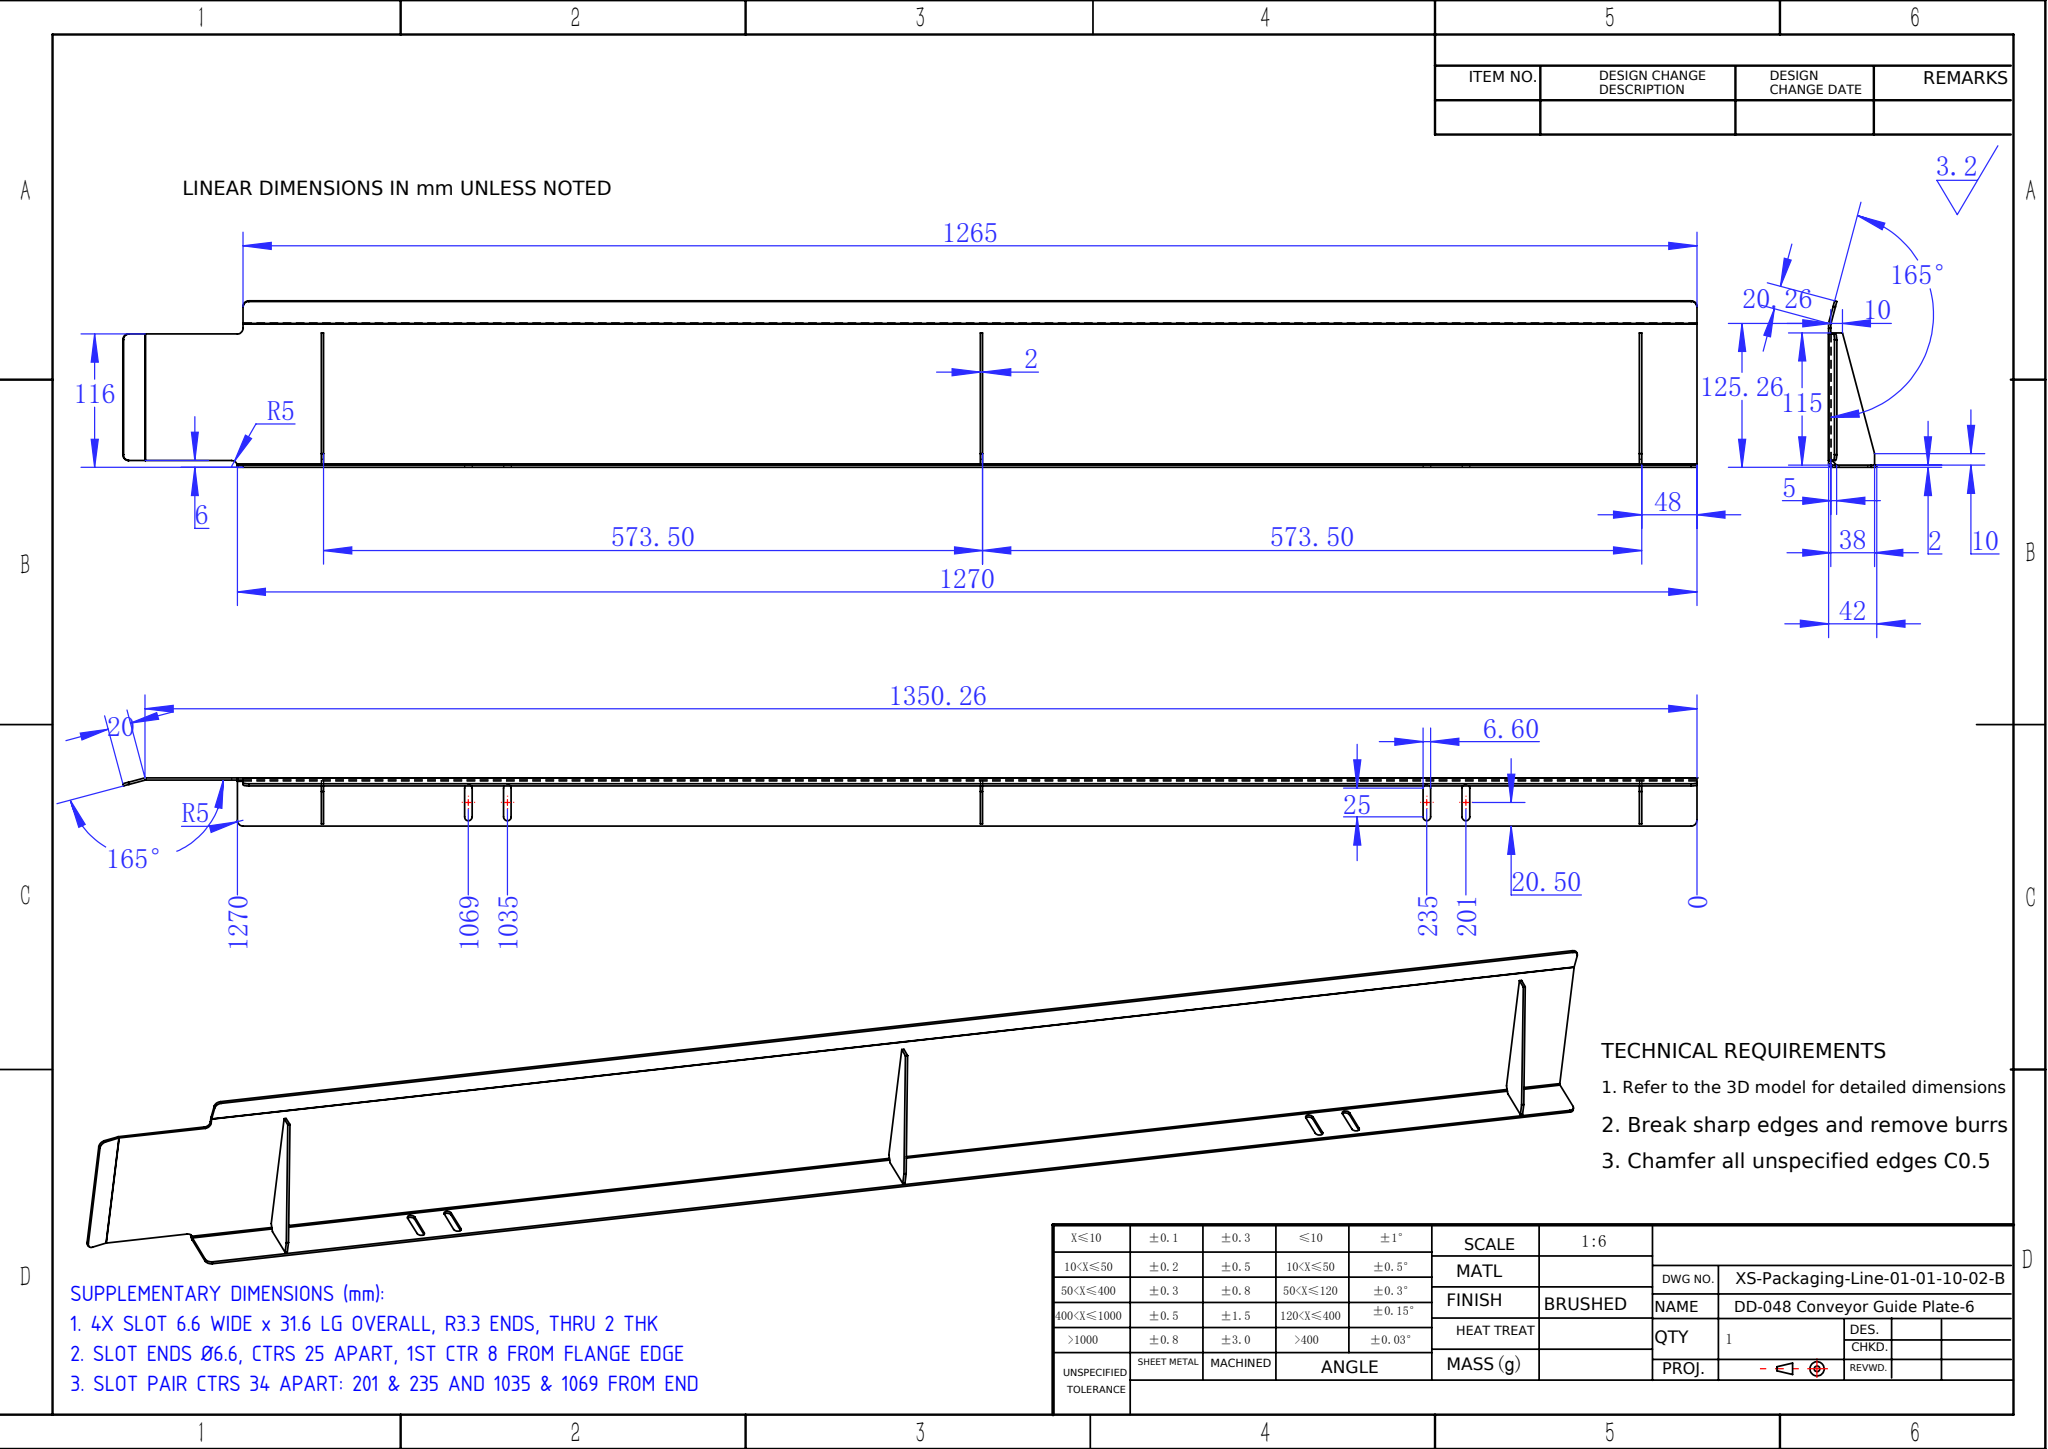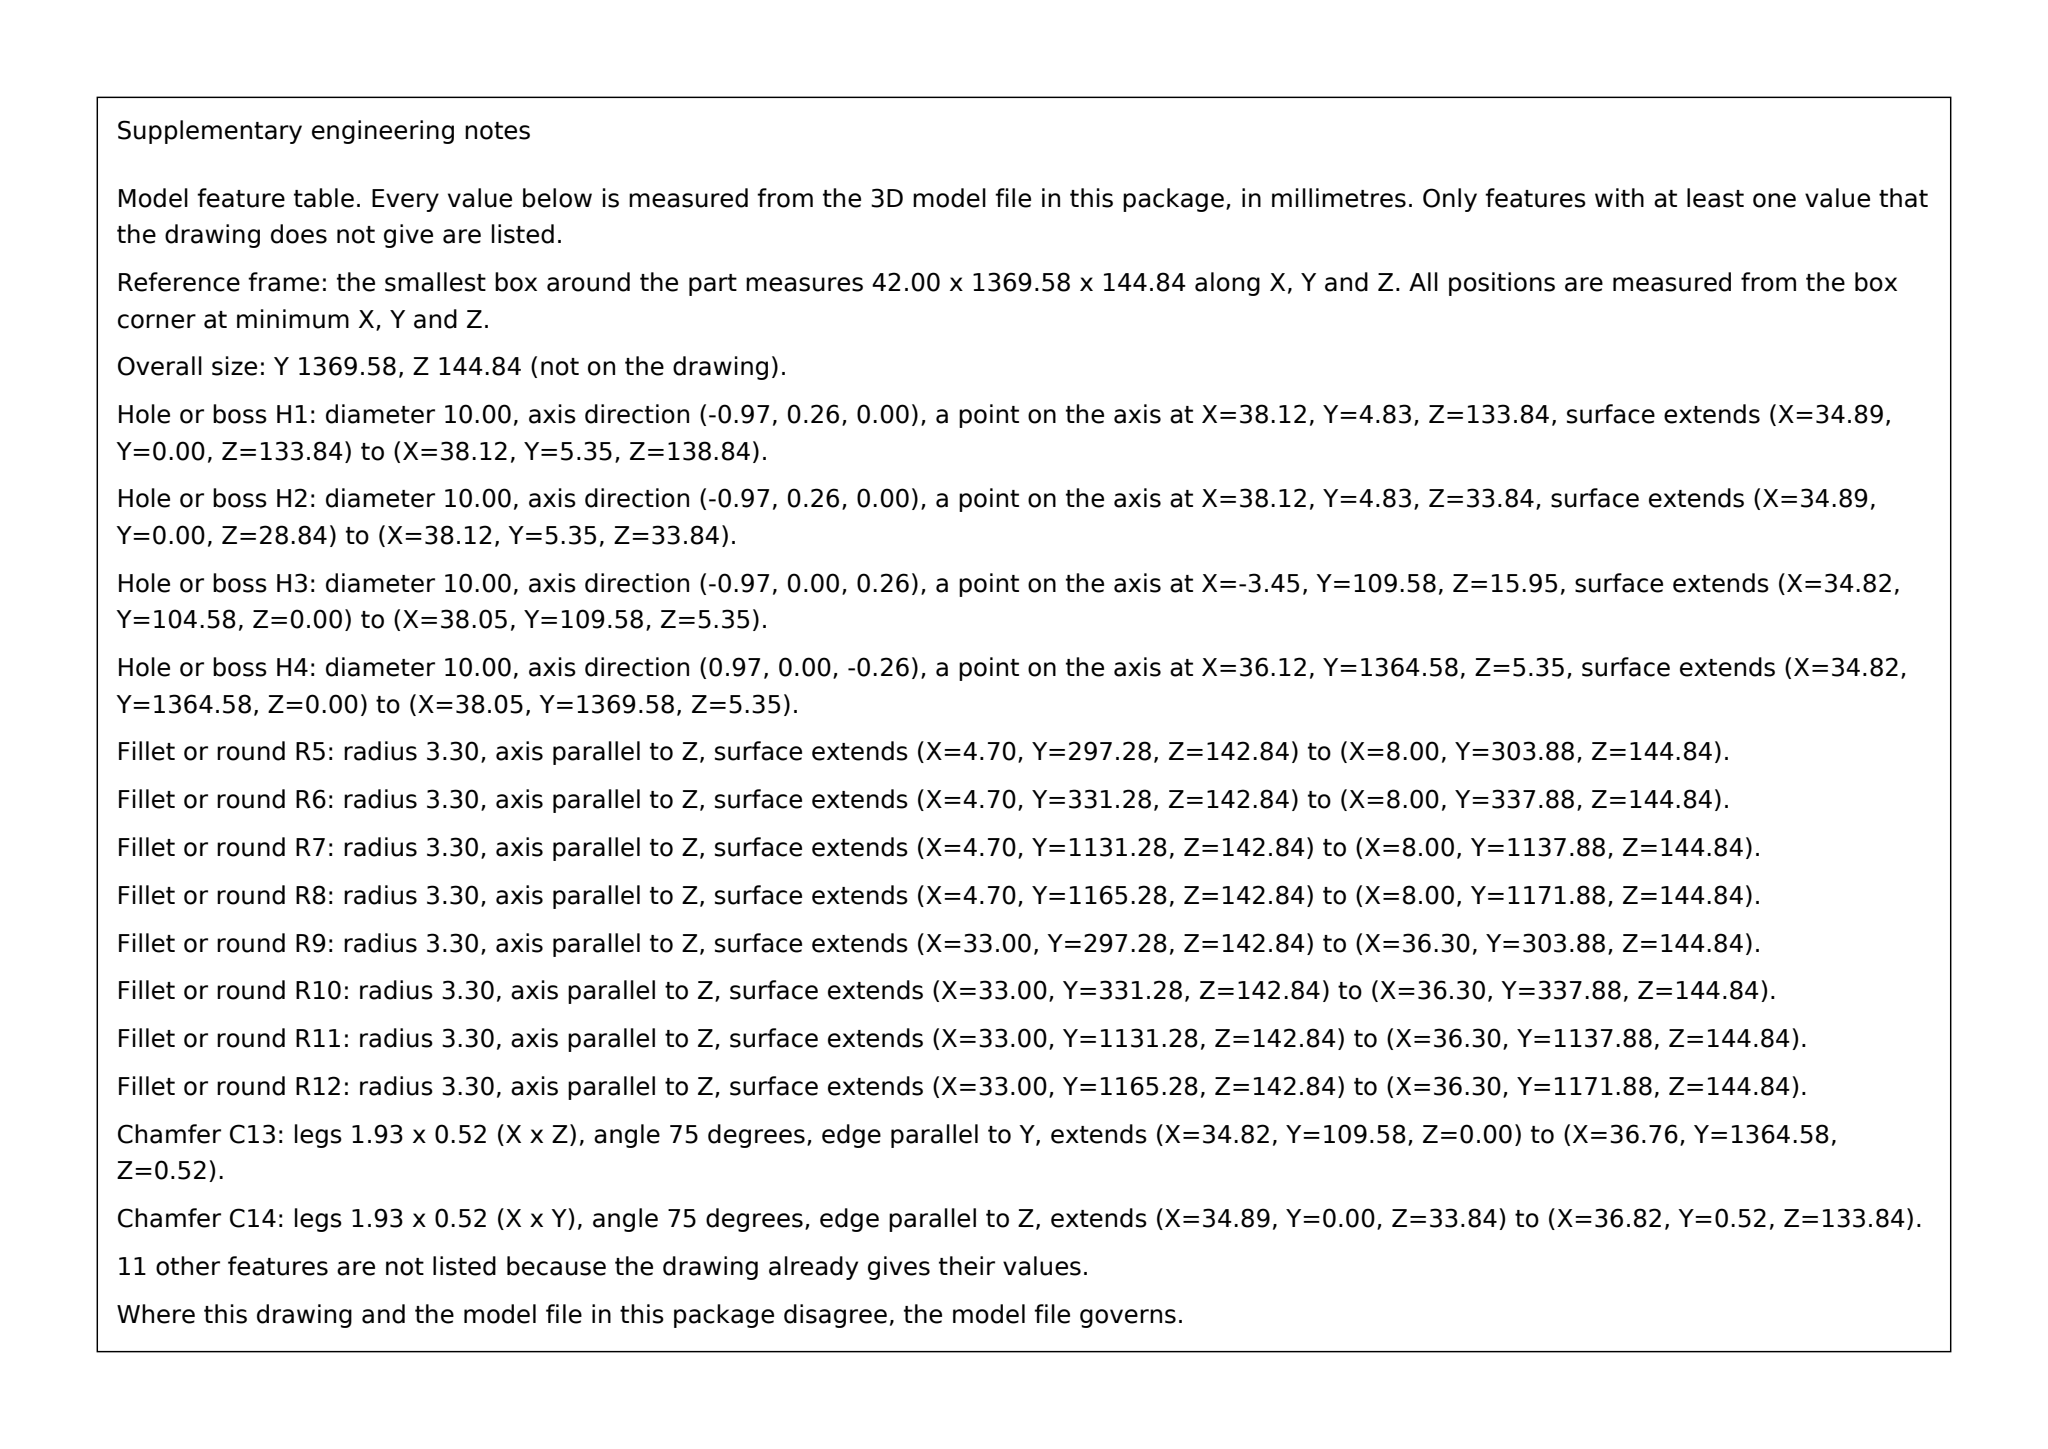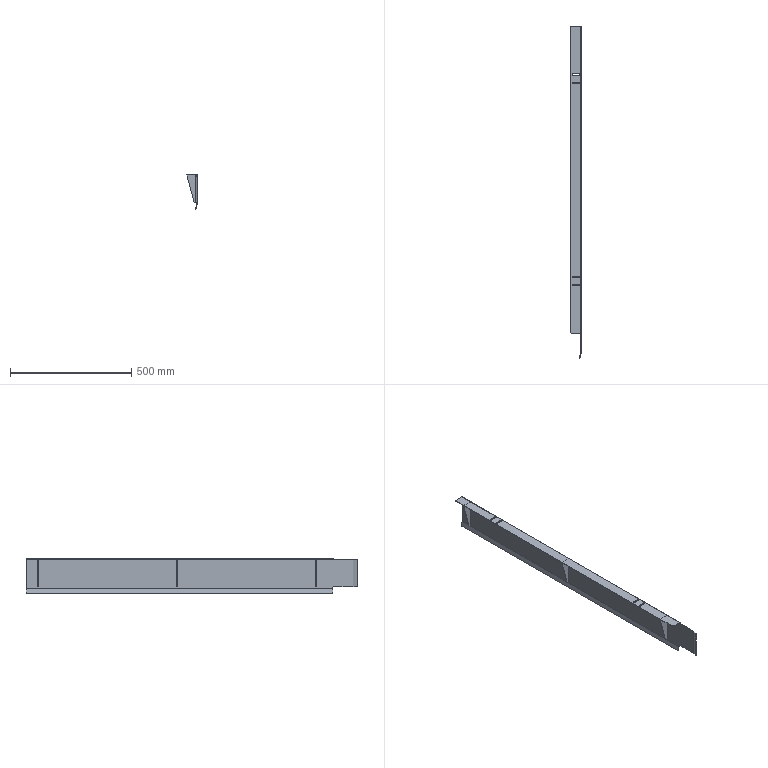Part | SolidWorks | mm | 1 solid | 77 faces | box 42 x 1369.58 x 144.84 mm | volume 505776 mm3 | plane 51 | cylinder 26 | commonest cylinder face diameters 6.6 x12 10 x8 2 x3 6 x3